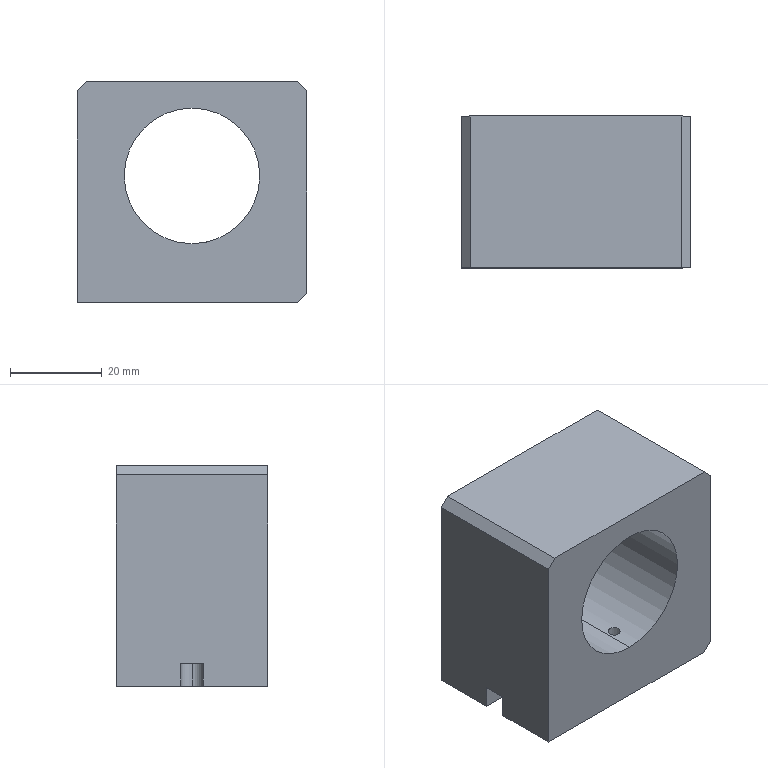Component | SolidWorks | H2020022-0435-1-1 | 1 solid | 64 faces | box 50 x 33 x 48 mm | volume 53798 mm3 | cylinder 28 | cone 24 | plane 12 | commonest cylinder face diameters 4.2 x20 2.5 x4 5 x2 29.5 x2 | material 6061 Aluminum Alloy
build123d program:
from build123d import *

# Parameters (mm, degrees)
SKETCH1_W             = 48
SKETCH1_H             = 50
BOSS_EXTRUDE1_DEPTH   = 33
SKETCH2_R             = 14.75
CUT_EXTRUDE1_DEPTH    = 48.854
M5_TAPPED_HOLE1_D     = 4.2
M5_TAPPED_HOLE1_DEPTH = 12.4
M5_TAPPED_HOLE1_TIP   = 1.262
CUT_EXTRUDE2_DEPTH    = 5
CIRPATTERN1_COUNT     = 8
CHAMFER1_SIZE         = 2
M3_TAPPED_HOLE1_D     = 2.5
M3_TAPPED_HOLE1_DEPTH = 7.5
M3_TAPPED_HOLE1_TIP   = 0.7511


with BuildPart() as part:
    # Sketch1 → Boss-Extrude1 (new body)
    with BuildSketch(Plane.XY):
        Rectangle(SKETCH1_W, SKETCH1_H)
    extrude(amount=BOSS_EXTRUDE1_DEPTH)

    # Sketch2 → Cut-Extrude1 (cut, through all)
    with BuildSketch(Plane.XY.offset(33)):
        with Locations((3.5, 0)):
            Circle(SKETCH2_R)
    extrude(amount=-CUT_EXTRUDE1_DEPTH, mode=Mode.SUBTRACT)

    # M5 Tapped Hole1
    with Locations(Plane.ZY.offset(24)):
        with Locations((6.5, -2), (6.5, 20), (26.5, 20), (26.5, -2)):
            Hole(M5_TAPPED_HOLE1_D / 2, depth=M5_TAPPED_HOLE1_DEPTH)
            with Locations((0, 0, -(M5_TAPPED_HOLE1_DEPTH + M5_TAPPED_HOLE1_TIP / 2))):  # 118° drill point
                Cone(0, M5_TAPPED_HOLE1_D / 2, M5_TAPPED_HOLE1_TIP, mode=Mode.SUBTRACT)

    # Sketch5 → Cut-Extrude2 (cut)
    with BuildSketch(Plane.ZY.offset(24)):
        with BuildLine():
            Line((19, 25), (19, -5))
            ThreePointArc((19, -5), (16.5, -7.5), (14, -5))
            Line((14, -5), (14, 25))
            ThreePointArc((14, 25), (16.5, 27.5), (19, 25))
        make_face()
    extrude(amount=-CUT_EXTRUDE2_DEPTH, mode=Mode.SUBTRACT)

    # Sketch9 → M5 Tapped Hole2 (revolve, cut)
    with BuildSketch(Plane(origin=(16.935, 13.435, 0), x_dir=(0, 1, 0), z_dir=(1, 0, 0))):
        Polygon((0, 0), (0, 13.662), (2.1, 12.4), (2.1, 0), align=None)
    m5_tapped_hole2 = revolve(axis=Axis((16.935, 13.435, -6.35), (0, 0, 1)), mode=Mode.SUBTRACT)

    # CirPattern1: M5 Tapped Hole2 ×8 about axis, 2 skipped
    cirpattern1_axis = Axis((3.5, 0, 0), (0, 0, 1))
    add([m5_tapped_hole2.rotate(cirpattern1_axis, i * 360 / CIRPATTERN1_COUNT) for i in range(1, CIRPATTERN1_COUNT) if i not in (3, 7)], mode=Mode.SUBTRACT)

    # Chamfer1
    chamfer1_edges = [part.edges().sort_by_distance(p)[0] for p in [
        (24, -25, 16.5),
        (-24, -25, 16.5),
        (24, 25, 16.5),
    ]]
    chamfer(chamfer1_edges, length=CHAMFER1_SIZE)

    # M3 Tapped Hole1
    with Locations(Plane(origin=(0, -25, 0), x_dir=(-1, 0, 0), z_dir=(0, -1, 0))):
        with Locations((14, -4), (14, -14)):
            Hole(M3_TAPPED_HOLE1_D / 2, depth=M3_TAPPED_HOLE1_DEPTH)
            with Locations((0, 0, -(M3_TAPPED_HOLE1_DEPTH + M3_TAPPED_HOLE1_TIP / 2))):  # 118° drill point
                Cone(0, M3_TAPPED_HOLE1_D / 2, M3_TAPPED_HOLE1_TIP, mode=Mode.SUBTRACT)


solid = part.part

# Placed as in the assembly
solid = solid.moved(Location((3.932, 8.813, 414.197), (90, 0, 90)))